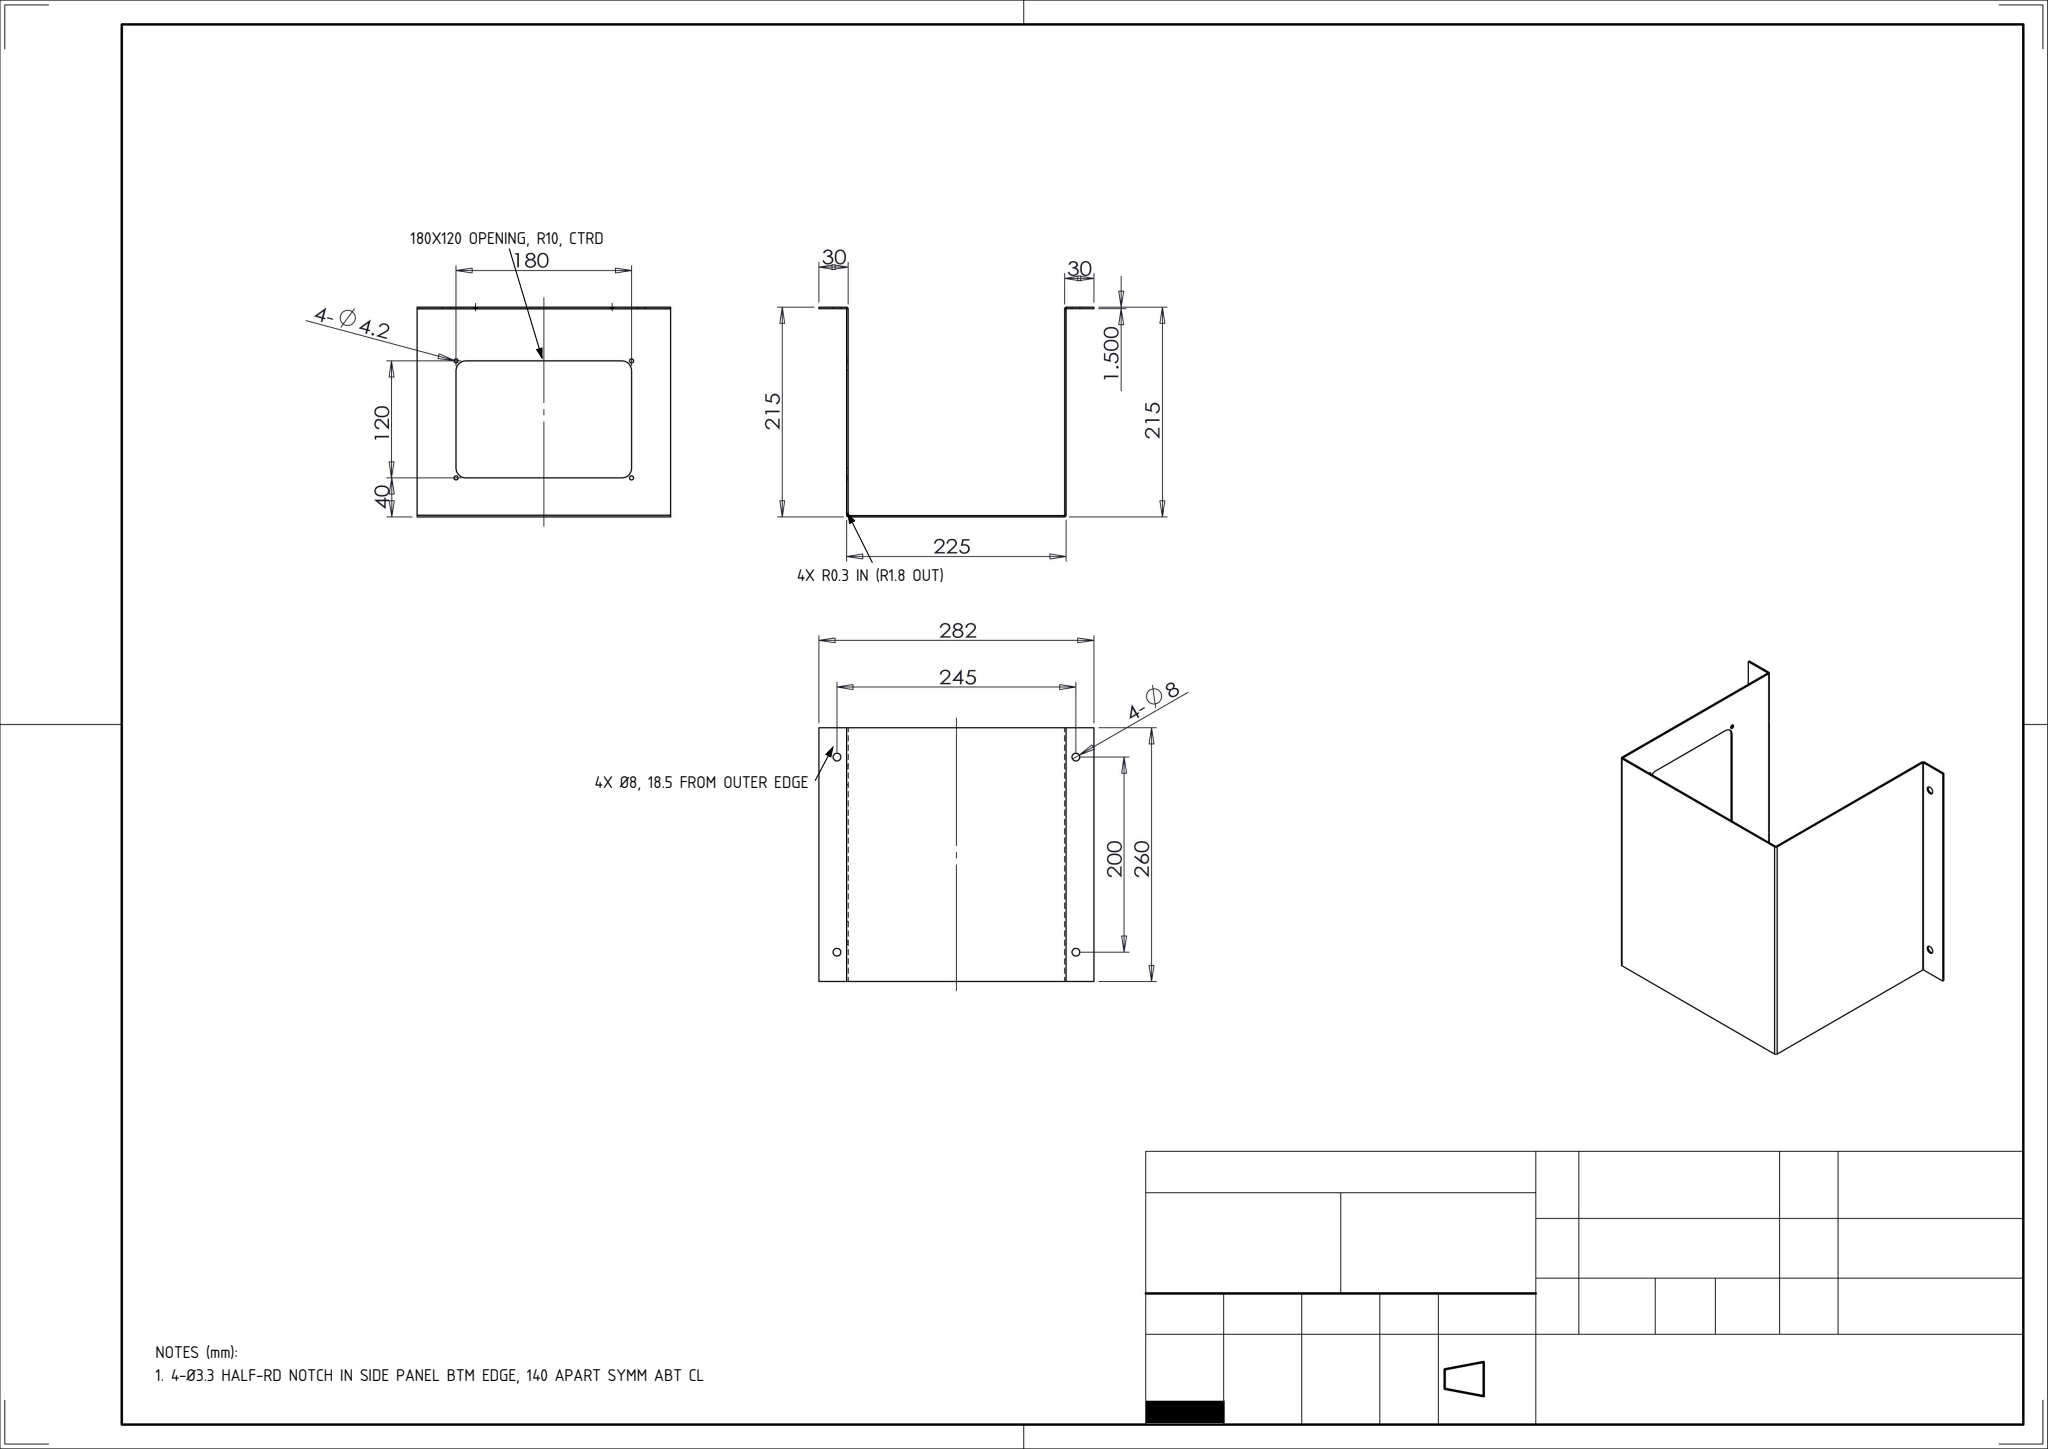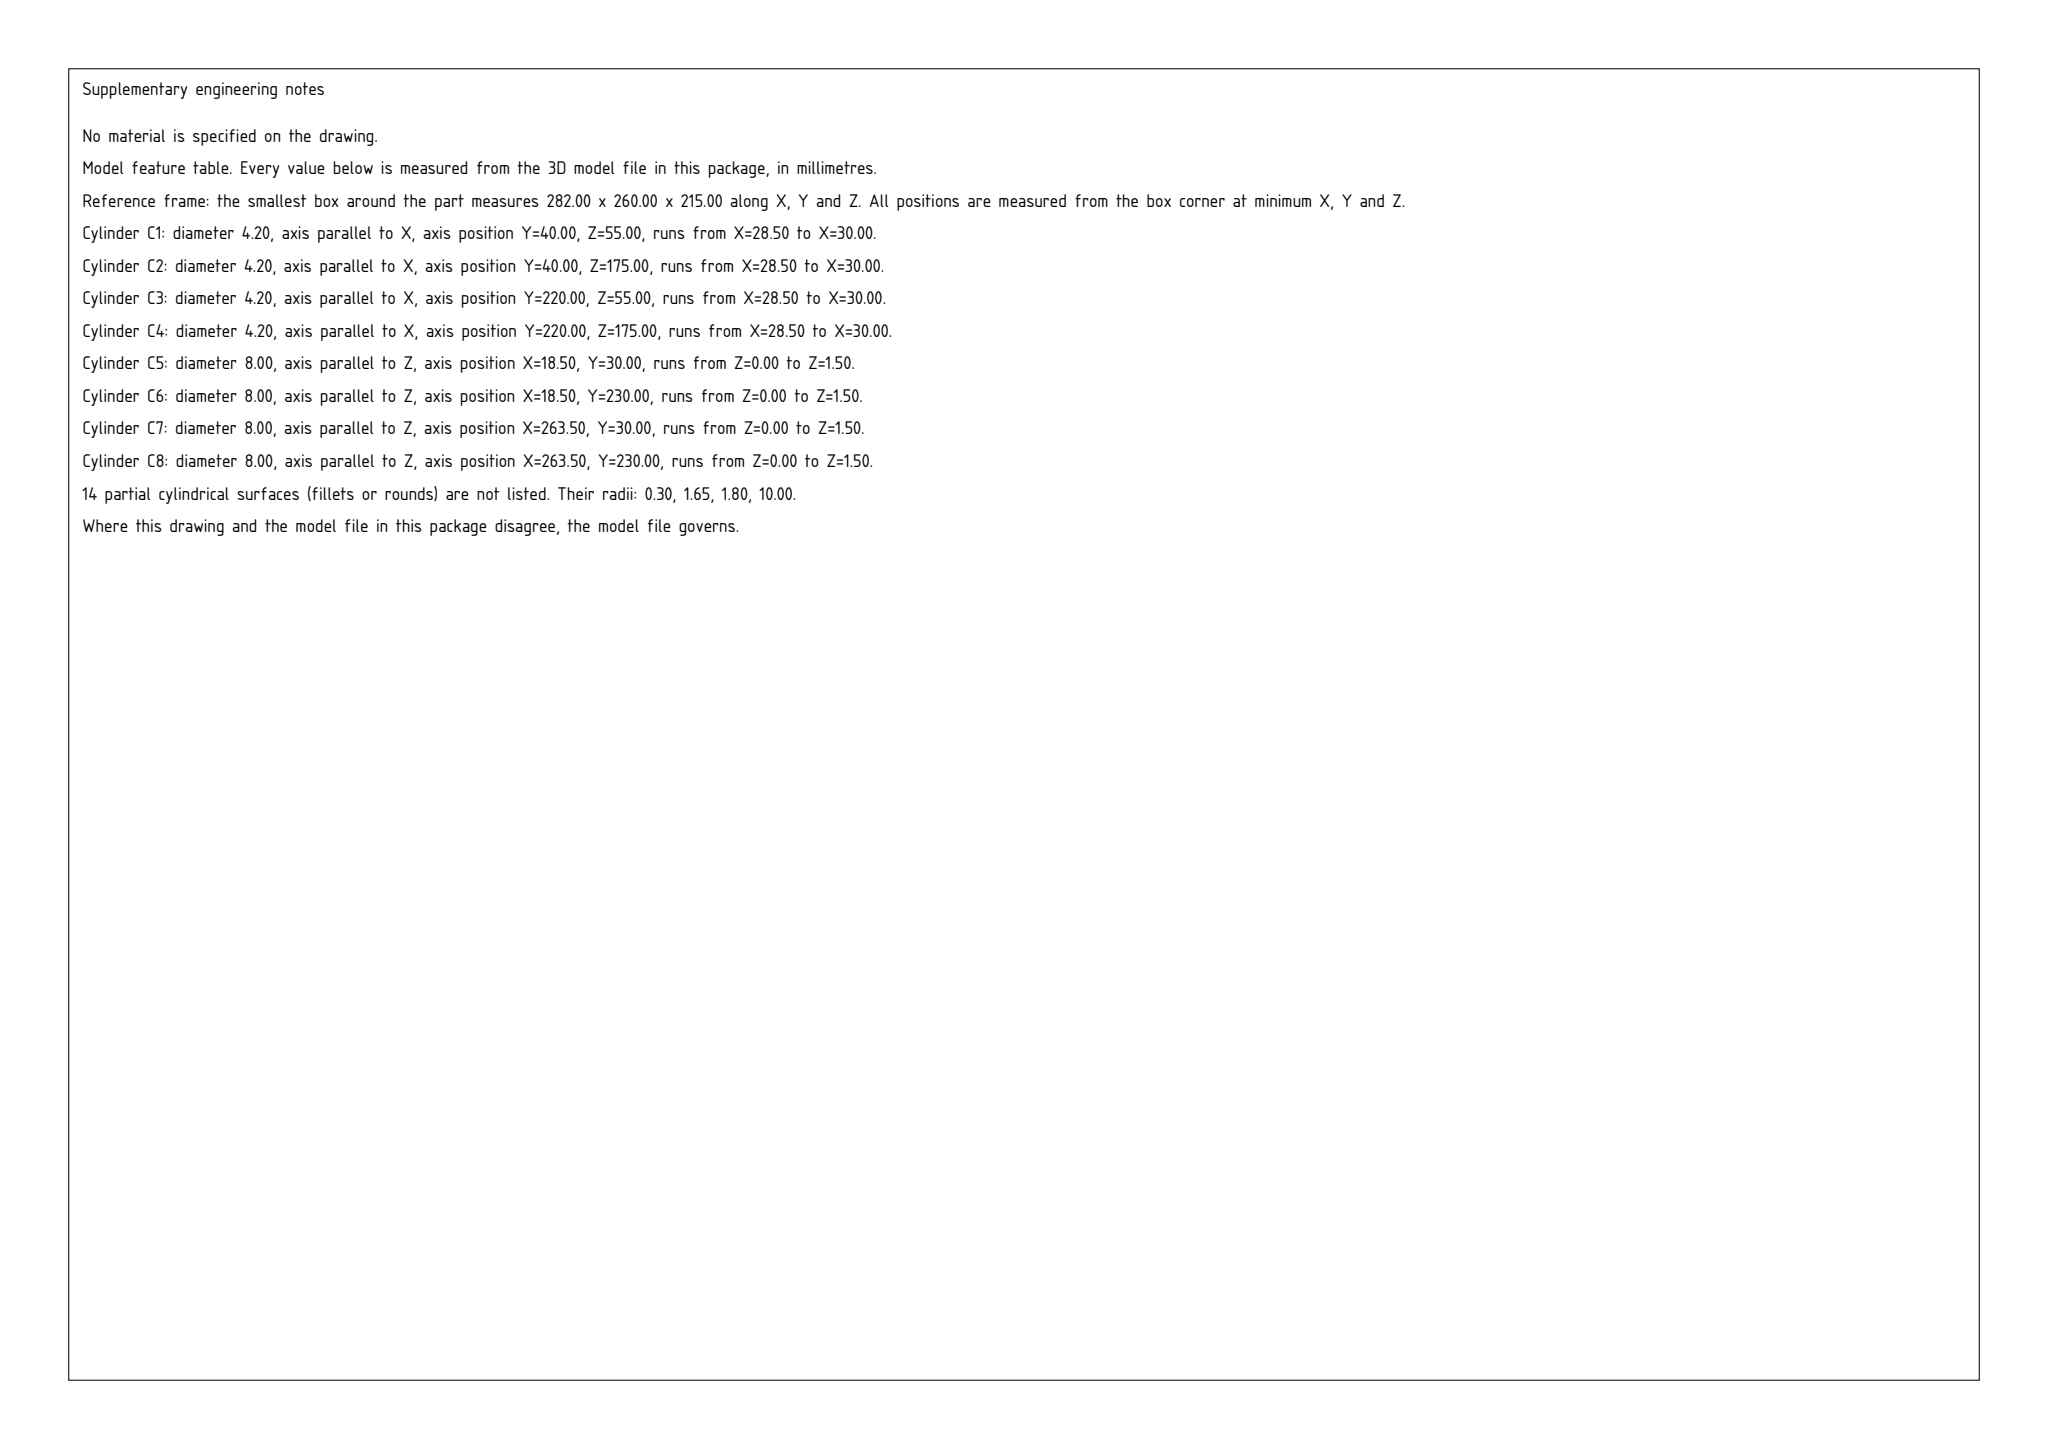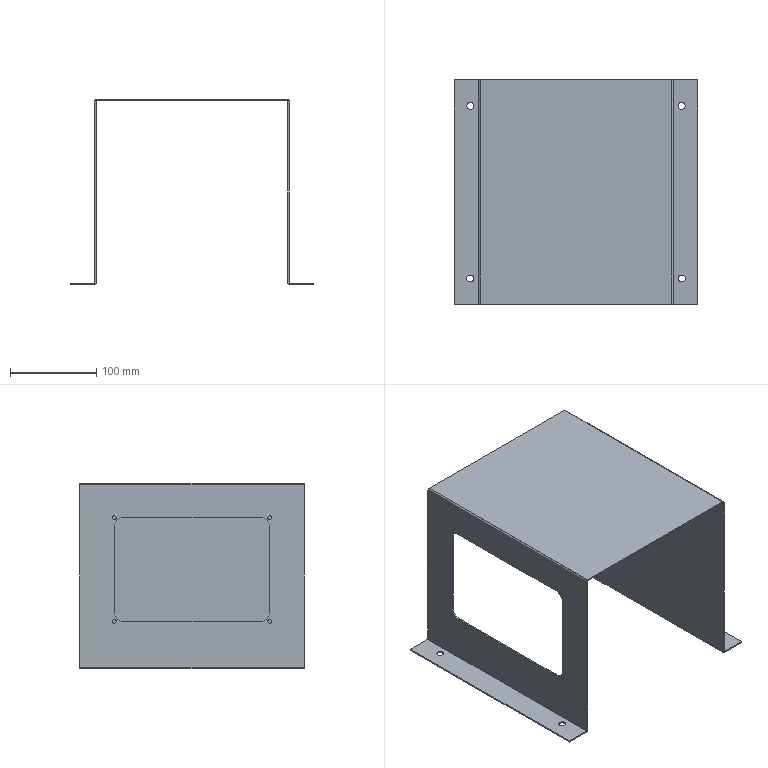Part | SolidWorks | mm | 1 solid | 68 faces | box 282 x 260 x 215 mm | volume 243142 mm3 | plane 36 | cylinder 32 | commonest cylinder face diameters 4.2 x8 8 x8 3.3 x4 3.6 x4 0.6 x4 20 x4
Drawing notes:
OPENING 180 W X 120 H, R10 CORNERS, CTRD ON 260 DEPTH | from the solid: x-normal cut bounded by y=40/220 (180) and z=55/175 (120); four Ø20 x-axis cyls at (y,z)=(50,65),(50,165),(210,65),(210,165) = R10 corners; centred in 260
4-Ø3.3 HALF-RD NOTCH IN SIDE PANEL BTM EDGE, 140 APART SYMM ABT CL | from the solid: Ø3.3 x-axis cyls L1.49 (=1.5 wall) at (y=60,z=0) x2 and (y=200,z=0) x2; z=0 bottom edge; 60 & 200 = 70 each side of 130 CL
4-Ø8 IN 30 FLANGES: 18.5 FROM OUTER EDGE, 245 BETWEEN CTRS | from the solid: Ø8 z-axis holes at x=18.5 and x=263.5; flange edges x=0 and x=282 -> 18.5 edge dist; 263.5-18.5=245
UNSPECIFIED BEND RADII R0.3 INSIDE (R1.8 OUTSIDE), 4 PLCS | from the solid: Ø0.6 and Ø3.6 y-axis cyls L260 at (28.2,1.8),(30.3,213.2),(251.7,213.2),(253.8,1.8) = inner R0.3 / outer R1.8 over 1.5 thk